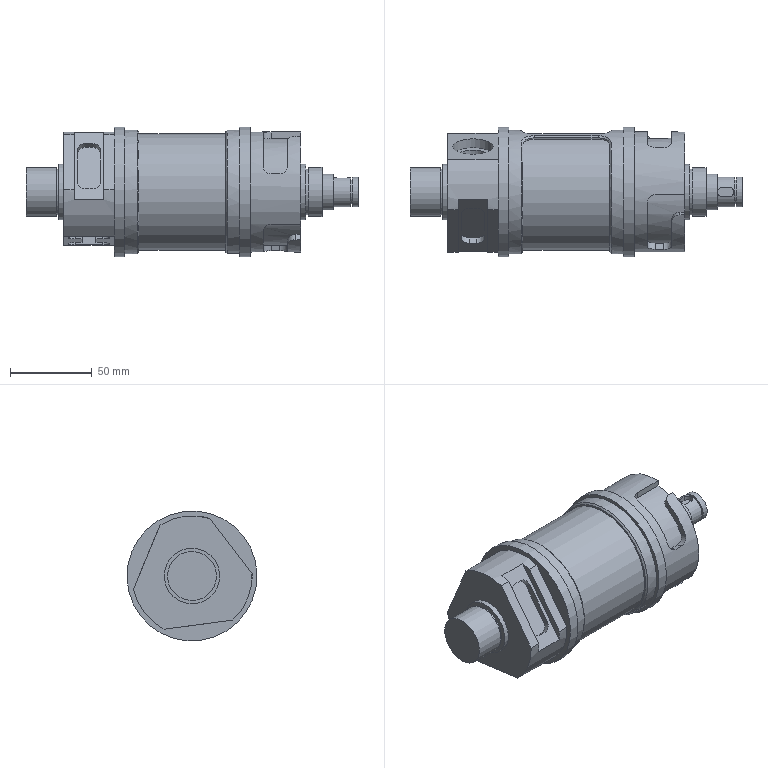Component | NX | DRIVEN_SHAFT | 1 solid | 126 faces | volume 607914 mm3 | plane 65 | cylinder 49 | spline 12 | commonest cylinder face diameters 10 x16 8 x8 73.5 x4 18 x3 65.5 x3 30 x2 28 x2 34 x2